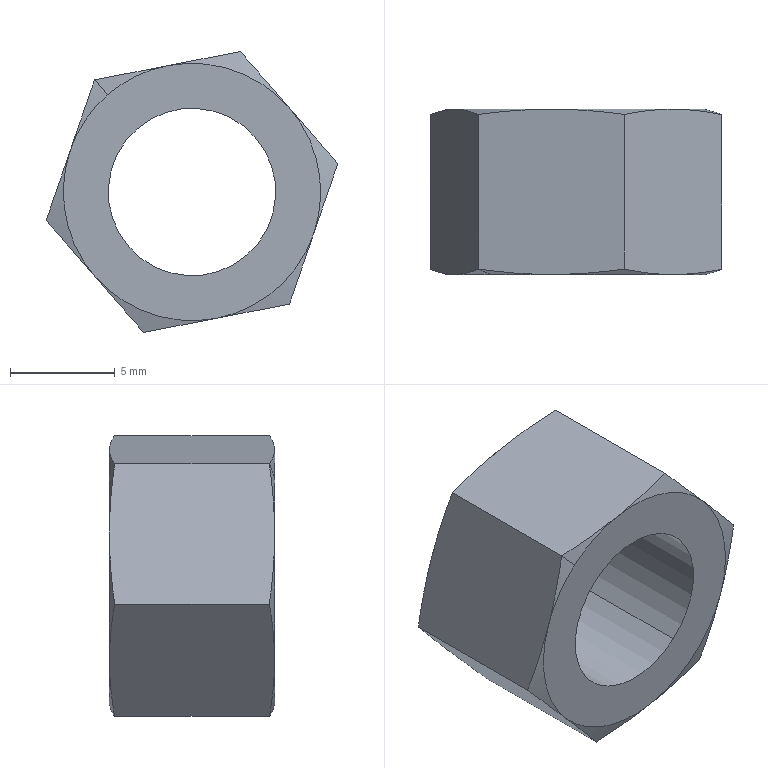Component | SolidWorks | GB_T41-2000Type1HexNutGradeCM8-1 | 1 solid | 24 faces | box 13.94 x 7.9 x 13.43 mm | volume 636 mm3 | cone 14 | plane 8 | cylinder 2 | commonest cylinder face diameters 8 x2
STEP:
#1=COLOUR_RGB('',0.7922,0.8196,0.9333);
#2=FILL_AREA_STYLE_COLOUR('',#1);
#3=FILL_AREA_STYLE('',(#2));
#4=SURFACE_STYLE_FILL_AREA(#3);
#5=SURFACE_SIDE_STYLE('',(#4));
#6=SURFACE_STYLE_USAGE(.BOTH.,#5);
#7=PRESENTATION_STYLE_ASSIGNMENT((#6));
#8=CARTESIAN_POINT('',(2.999,-2.205,10.51));
#9=VERTEX_POINT('',#8);
#10=CARTESIAN_POINT('',(3.112,-2.205,10.565));
#11=VERTEX_POINT('',#10);
#12=CARTESIAN_POINT('',(2.953,-2.205,10.748));
#13=DIRECTION('',(0.,-1.,-0.));
#14=DIRECTION('',(-0.656,-0.,0.7547));
#15=AXIS2_PLACEMENT_3D('',#12,#13,#14);
#16=CIRCLE('',#15,0.2421);
#17=EDGE_CURVE('',#9,#11,#16,.T.);
#18=ORIENTED_EDGE('',*,*,#17,.T.);
#19=CARTESIAN_POINT('',(3.136,-2.215,10.537));
#20=VERTEX_POINT('',#19);
#21=CARTESIAN_POINT('',(3.112,-2.205,10.565));
#22=DIRECTION('',(0.6337,-0.2588,-0.729));
#23=VECTOR('',#22,39.37);
#24=LINE('',#21,#23);
#25=EDGE_CURVE('',#11,#20,#24,.T.);
#26=ORIENTED_EDGE('',*,*,#25,.T.);
#27=CARTESIAN_POINT('',(3.136,-2.215,10.537));
#28=CARTESIAN_POINT('',(3.091,-2.209,10.528));
#29=CARTESIAN_POINT('',(3.045,-2.205,10.519));
#30=CARTESIAN_POINT('',(2.999,-2.205,10.51));
#31=B_SPLINE_CURVE_WITH_KNOTS('',3,(#27,#28,#29,#30),.UNSPECIFIED.,.F.,.F.,(4,4),(0.,0.003559),.UNSPECIFIED.);
#32=EDGE_CURVE('',#20,#9,#31,.T.);
#33=ORIENTED_EDGE('',*,*,#32,.T.);
#34=EDGE_LOOP('',(#18,#26,#33));
#35=FACE_OUTER_BOUND('',#34,.T.);
#36=CARTESIAN_POINT('',(2.953,-2.205,10.748));
#37=DIRECTION('',(0.,-1.,-0.));
#38=DIRECTION('',(0.656,0.,-0.7547));
#39=AXIS2_PLACEMENT_3D('',#36,#37,#38);
#40=CONICAL_SURFACE('',#39,0.2421,1.309);
#41=ADVANCED_FACE('',(#35),#40,.T.);
#42=CARTESIAN_POINT('',(2.794,-2.516,10.931));
#43=VERTEX_POINT('',#42);
#44=CARTESIAN_POINT('',(2.724,-2.516,10.827));
#45=VERTEX_POINT('',#44);
#46=CARTESIAN_POINT('',(2.953,-2.516,10.748));
#47=DIRECTION('',(0.,-1.,-0.));
#48=DIRECTION('',(-0.656,0.,0.7547));
#49=AXIS2_PLACEMENT_3D('',#46,#47,#48);
#50=CIRCLE('',#49,0.2421);
#51=EDGE_CURVE('',#43,#45,#50,.T.);
#52=ORIENTED_EDGE('',*,*,#51,.F.);
#53=CARTESIAN_POINT('',(2.769,-2.506,10.959));
#54=VERTEX_POINT('',#53);
#55=CARTESIAN_POINT('',(2.794,-2.516,10.931));
#56=DIRECTION('',(-0.6337,0.2588,0.729));
#57=VECTOR('',#56,39.37);
#58=LINE('',#55,#57);
#59=EDGE_CURVE('',#43,#54,#58,.T.);
#60=ORIENTED_EDGE('',*,*,#59,.T.);
#61=CARTESIAN_POINT('',(2.769,-2.506,10.959));
#62=CARTESIAN_POINT('',(2.754,-2.512,10.915));
#63=CARTESIAN_POINT('',(2.739,-2.516,10.871));
#64=CARTESIAN_POINT('',(2.724,-2.516,10.827));
#65=B_SPLINE_CURVE_WITH_KNOTS('',3,(#61,#62,#63,#64),.UNSPECIFIED.,.F.,.F.,(4,4),(0.,0.003559),.UNSPECIFIED.);
#66=EDGE_CURVE('',#54,#45,#65,.T.);
#67=ORIENTED_EDGE('',*,*,#66,.T.);
#68=EDGE_LOOP('',(#52,#60,#67));
#69=FACE_OUTER_BOUND('',#68,.T.);
#70=CARTESIAN_POINT('',(2.953,-2.516,10.748));
#71=DIRECTION('',(-0.,1.,0.));
#72=DIRECTION('',(-0.656,0.,0.7547));
#73=AXIS2_PLACEMENT_3D('',#70,#71,#72);
#74=CONICAL_SURFACE('',#73,0.2421,1.309);
#75=ADVANCED_FACE('',(#69),#74,.T.);
#76=CARTESIAN_POINT('',(2.849,-2.205,10.867));
#77=VERTEX_POINT('',#76);
#78=CARTESIAN_POINT('',(3.056,-2.205,10.629));
#79=VERTEX_POINT('',#78);
#80=CARTESIAN_POINT('',(2.953,-2.205,10.748));
#81=DIRECTION('',(-0.,1.,0.));
#82=DIRECTION('',(0.656,0.,-0.7547));
#83=AXIS2_PLACEMENT_3D('',#80,#81,#82);
#84=CIRCLE('',#83,0.1575);
#85=EDGE_CURVE('',#77,#79,#84,.T.);
#86=ORIENTED_EDGE('',*,*,#85,.T.);
#87=CARTESIAN_POINT('',(3.056,-2.516,10.629));
#88=VERTEX_POINT('',#87);
#89=CARTESIAN_POINT('',(3.056,-2.205,10.629));
#90=DIRECTION('',(0.,-1.,-0.));
#91=VECTOR('',#90,39.37);
#92=LINE('',#89,#91);
#93=EDGE_CURVE('',#79,#88,#92,.T.);
#94=ORIENTED_EDGE('',*,*,#93,.T.);
#95=CARTESIAN_POINT('',(2.849,-2.516,10.867));
#96=VERTEX_POINT('',#95);
#97=CARTESIAN_POINT('',(2.953,-2.516,10.748));
#98=DIRECTION('',(-0.,1.,0.));
#99=DIRECTION('',(0.656,0.,-0.7547));
#100=AXIS2_PLACEMENT_3D('',#97,#98,#99);
#101=CIRCLE('',#100,0.1575);
#102=EDGE_CURVE('',#96,#88,#101,.T.);
#103=ORIENTED_EDGE('',*,*,#102,.F.);
#104=CARTESIAN_POINT('',(2.849,-2.205,10.867));
#105=DIRECTION('',(0.,-1.,-0.));
#106=VECTOR('',#105,39.37);
#107=LINE('',#104,#106);
#108=EDGE_CURVE('',#77,#96,#107,.T.);
#109=ORIENTED_EDGE('',*,*,#108,.F.);
#110=EDGE_LOOP('',(#86,#94,#103,#109));
#111=FACE_OUTER_BOUND('',#110,.T.);
#112=CARTESIAN_POINT('',(2.953,-2.205,10.748));
#113=DIRECTION('',(0.,-1.,-0.));
#114=DIRECTION('',(-0.656,-0.,0.7547));
#115=AXIS2_PLACEMENT_3D('',#112,#113,#114);
#116=CYLINDRICAL_SURFACE('',#115,0.1575);
#117=ADVANCED_FACE('',(#111),#116,.F.);
#118=CARTESIAN_POINT('',(2.77,-2.205,10.589));
#119=VERTEX_POINT('',#118);
#120=CARTESIAN_POINT('',(2.678,-2.215,10.695));
#121=VERTEX_POINT('',#120);
#122=CARTESIAN_POINT('',(2.77,-2.205,10.589));
#123=CARTESIAN_POINT('',(2.739,-2.205,10.625));
#124=CARTESIAN_POINT('',(2.709,-2.209,10.66));
#125=CARTESIAN_POINT('',(2.678,-2.215,10.695));
#126=B_SPLINE_CURVE_WITH_KNOTS('',3,(#122,#123,#124,#125),.UNSPECIFIED.,.F.,.F.,(4,4),(0.,0.003559),.UNSPECIFIED.);
#127=EDGE_CURVE('',#119,#121,#126,.T.);
#128=ORIENTED_EDGE('',*,*,#127,.T.);
#129=CARTESIAN_POINT('',(2.724,-2.205,10.827));
#130=VERTEX_POINT('',#129);
#131=CARTESIAN_POINT('',(2.678,-2.215,10.695));
#132=CARTESIAN_POINT('',(2.693,-2.209,10.739));
#133=CARTESIAN_POINT('',(2.709,-2.205,10.783));
#134=CARTESIAN_POINT('',(2.724,-2.205,10.827));
#135=B_SPLINE_CURVE_WITH_KNOTS('',3,(#131,#132,#133,#134),.UNSPECIFIED.,.F.,.F.,(4,4),(0.,0.003559),.UNSPECIFIED.);
#136=EDGE_CURVE('',#121,#130,#135,.T.);
#137=ORIENTED_EDGE('',*,*,#136,.T.);
#138=CARTESIAN_POINT('',(2.953,-2.205,10.748));
#139=DIRECTION('',(0.,-1.,-0.));
#140=DIRECTION('',(-0.656,-0.,0.7547));
#141=AXIS2_PLACEMENT_3D('',#138,#139,#140);
#142=CIRCLE('',#141,0.2421);
#143=EDGE_CURVE('',#130,#119,#142,.T.);
#144=ORIENTED_EDGE('',*,*,#143,.T.);
#145=EDGE_LOOP('',(#128,#137,#144));
#146=FACE_OUTER_BOUND('',#145,.T.);
#147=CARTESIAN_POINT('',(2.953,-2.205,10.748));
#148=DIRECTION('',(0.,-1.,-0.));
#149=DIRECTION('',(0.656,0.,-0.7547));
#150=AXIS2_PLACEMENT_3D('',#147,#148,#149);
#151=CONICAL_SURFACE('',#150,0.2421,1.309);
#152=ADVANCED_FACE('',(#146),#151,.T.);
#153=CARTESIAN_POINT('',(2.862,-2.215,10.484));
#154=VERTEX_POINT('',#153);
#155=CARTESIAN_POINT('',(2.999,-2.205,10.51));
#156=CARTESIAN_POINT('',(2.953,-2.205,10.501));
#157=CARTESIAN_POINT('',(2.907,-2.209,10.493));
#158=CARTESIAN_POINT('',(2.862,-2.215,10.484));
#159=B_SPLINE_CURVE_WITH_KNOTS('',3,(#155,#156,#157,#158),.UNSPECIFIED.,.F.,.F.,(4,4),(0.,0.003559),.UNSPECIFIED.);
#160=EDGE_CURVE('',#9,#154,#159,.T.);
#161=ORIENTED_EDGE('',*,*,#160,.T.);
#162=CARTESIAN_POINT('',(2.862,-2.215,10.484));
#163=CARTESIAN_POINT('',(2.831,-2.209,10.519));
#164=CARTESIAN_POINT('',(2.801,-2.205,10.554));
#165=CARTESIAN_POINT('',(2.77,-2.205,10.589));
#166=B_SPLINE_CURVE_WITH_KNOTS('',3,(#162,#163,#164,#165),.UNSPECIFIED.,.F.,.F.,(4,4),(0.,0.003559),.UNSPECIFIED.);
#167=EDGE_CURVE('',#154,#119,#166,.T.);
#168=ORIENTED_EDGE('',*,*,#167,.T.);
#169=CARTESIAN_POINT('',(2.953,-2.205,10.748));
#170=DIRECTION('',(-0.,1.,0.));
#171=DIRECTION('',(0.656,0.,-0.7547));
#172=AXIS2_PLACEMENT_3D('',#169,#170,#171);
#173=CIRCLE('',#172,0.2421);
#174=EDGE_CURVE('',#9,#119,#173,.T.);
#175=ORIENTED_EDGE('',*,*,#174,.F.);
#176=EDGE_LOOP('',(#161,#168,#175));
#177=FACE_OUTER_BOUND('',#176,.T.);
#178=CARTESIAN_POINT('',(2.953,-2.205,10.748));
#179=DIRECTION('',(0.,-1.,-0.));
#180=DIRECTION('',(0.656,0.,-0.7547));
#181=AXIS2_PLACEMENT_3D('',#178,#179,#180);
#182=CONICAL_SURFACE('',#181,0.2421,1.309);
#183=ADVANCED_FACE('',(#177),#182,.T.);
#184=CARTESIAN_POINT('',(3.135,-2.205,10.907));
#185=VERTEX_POINT('',#184);
#186=CARTESIAN_POINT('',(3.227,-2.215,10.801));
#187=VERTEX_POINT('',#186);
#188=CARTESIAN_POINT('',(3.135,-2.205,10.907));
#189=CARTESIAN_POINT('',(3.166,-2.205,10.871));
#190=CARTESIAN_POINT('',(3.197,-2.209,10.836));
#191=CARTESIAN_POINT('',(3.227,-2.215,10.801));
#192=B_SPLINE_CURVE_WITH_KNOTS('',3,(#188,#189,#190,#191),.UNSPECIFIED.,.F.,.F.,(4,4),(0.,0.003559),.UNSPECIFIED.);
#193=EDGE_CURVE('',#185,#187,#192,.T.);
#194=ORIENTED_EDGE('',*,*,#193,.T.);
#195=CARTESIAN_POINT('',(3.182,-2.205,10.669));
#196=VERTEX_POINT('',#195);
#197=CARTESIAN_POINT('',(3.227,-2.215,10.801));
#198=CARTESIAN_POINT('',(3.212,-2.209,10.758));
#199=CARTESIAN_POINT('',(3.197,-2.205,10.713));
#200=CARTESIAN_POINT('',(3.182,-2.205,10.669));
#201=B_SPLINE_CURVE_WITH_KNOTS('',3,(#197,#198,#199,#200),.UNSPECIFIED.,.F.,.F.,(4,4),(0.,0.003559),.UNSPECIFIED.);
#202=EDGE_CURVE('',#187,#196,#201,.T.);
#203=ORIENTED_EDGE('',*,*,#202,.T.);
#204=CARTESIAN_POINT('',(2.953,-2.205,10.748));
#205=DIRECTION('',(0.,-1.,-0.));
#206=DIRECTION('',(-0.656,-0.,0.7547));
#207=AXIS2_PLACEMENT_3D('',#204,#205,#206);
#208=CIRCLE('',#207,0.2421);
#209=EDGE_CURVE('',#196,#185,#208,.T.);
#210=ORIENTED_EDGE('',*,*,#209,.T.);
#211=EDGE_LOOP('',(#194,#203,#210));
#212=FACE_OUTER_BOUND('',#211,.T.);
#213=CARTESIAN_POINT('',(2.953,-2.205,10.748));
#214=DIRECTION('',(0.,-1.,-0.));
#215=DIRECTION('',(0.656,0.,-0.7547));
#216=AXIS2_PLACEMENT_3D('',#213,#214,#215);
#217=CONICAL_SURFACE('',#216,0.2421,1.309);
#218=ADVANCED_FACE('',(#212),#217,.T.);
#219=CARTESIAN_POINT('',(2.907,-2.205,10.986));
#220=VERTEX_POINT('',#219);
#221=CARTESIAN_POINT('',(3.044,-2.215,11.012));
#222=VERTEX_POINT('',#221);
#223=CARTESIAN_POINT('',(2.907,-2.205,10.986));
#224=CARTESIAN_POINT('',(2.953,-2.205,10.995));
#225=CARTESIAN_POINT('',(2.998,-2.209,11.003));
#226=CARTESIAN_POINT('',(3.044,-2.215,11.012));
#227=B_SPLINE_CURVE_WITH_KNOTS('',3,(#223,#224,#225,#226),.UNSPECIFIED.,.F.,.F.,(4,4),(0.,0.003559),.UNSPECIFIED.);
#228=EDGE_CURVE('',#220,#222,#227,.T.);
#229=ORIENTED_EDGE('',*,*,#228,.T.);
#230=CARTESIAN_POINT('',(3.044,-2.215,11.012));
#231=CARTESIAN_POINT('',(3.074,-2.209,10.977));
#232=CARTESIAN_POINT('',(3.105,-2.205,10.942));
#233=CARTESIAN_POINT('',(3.135,-2.205,10.907));
#234=B_SPLINE_CURVE_WITH_KNOTS('',3,(#230,#231,#232,#233),.UNSPECIFIED.,.F.,.F.,(4,4),(0.,0.003559),.UNSPECIFIED.);
#235=EDGE_CURVE('',#222,#185,#234,.T.);
#236=ORIENTED_EDGE('',*,*,#235,.T.);
#237=CARTESIAN_POINT('',(2.953,-2.205,10.748));
#238=DIRECTION('',(0.,-1.,-0.));
#239=DIRECTION('',(-0.656,-0.,0.7547));
#240=AXIS2_PLACEMENT_3D('',#237,#238,#239);
#241=CIRCLE('',#240,0.2421);
#242=EDGE_CURVE('',#185,#220,#241,.T.);
#243=ORIENTED_EDGE('',*,*,#242,.T.);
#244=EDGE_LOOP('',(#229,#236,#243));
#245=FACE_OUTER_BOUND('',#244,.T.);
#246=CARTESIAN_POINT('',(2.953,-2.205,10.748));
#247=DIRECTION('',(0.,-1.,-0.));
#248=DIRECTION('',(0.656,0.,-0.7547));
#249=AXIS2_PLACEMENT_3D('',#246,#247,#248);
#250=CONICAL_SURFACE('',#249,0.2421,1.309);
#251=ADVANCED_FACE('',(#245),#250,.T.);
#252=CARTESIAN_POINT('',(2.769,-2.215,10.959));
#253=VERTEX_POINT('',#252);
#254=CARTESIAN_POINT('',(2.724,-2.205,10.827));
#255=CARTESIAN_POINT('',(2.739,-2.205,10.871));
#256=CARTESIAN_POINT('',(2.754,-2.209,10.915));
#257=CARTESIAN_POINT('',(2.769,-2.215,10.959));
#258=B_SPLINE_CURVE_WITH_KNOTS('',3,(#254,#255,#256,#257),.UNSPECIFIED.,.F.,.F.,(4,4),(0.,0.003559),.UNSPECIFIED.);
#259=EDGE_CURVE('',#130,#253,#258,.T.);
#260=ORIENTED_EDGE('',*,*,#259,.T.);
#261=CARTESIAN_POINT('',(2.769,-2.215,10.959));
#262=CARTESIAN_POINT('',(2.815,-2.209,10.968));
#263=CARTESIAN_POINT('',(2.861,-2.205,10.977));
#264=CARTESIAN_POINT('',(2.907,-2.205,10.986));
#265=B_SPLINE_CURVE_WITH_KNOTS('',3,(#261,#262,#263,#264),.UNSPECIFIED.,.F.,.F.,(4,4),(0.,0.003559),.UNSPECIFIED.);
#266=EDGE_CURVE('',#253,#220,#265,.T.);
#267=ORIENTED_EDGE('',*,*,#266,.T.);
#268=CARTESIAN_POINT('',(2.953,-2.205,10.748));
#269=DIRECTION('',(0.,-1.,-0.));
#270=DIRECTION('',(-0.656,-0.,0.7547));
#271=AXIS2_PLACEMENT_3D('',#268,#269,#270);
#272=CIRCLE('',#271,0.2421);
#273=EDGE_CURVE('',#220,#130,#272,.T.);
#274=ORIENTED_EDGE('',*,*,#273,.T.);
#275=EDGE_LOOP('',(#260,#267,#274));
#276=FACE_OUTER_BOUND('',#275,.T.);
#277=CARTESIAN_POINT('',(2.953,-2.205,10.748));
#278=DIRECTION('',(0.,-1.,-0.));
#279=DIRECTION('',(0.656,0.,-0.7547));
#280=AXIS2_PLACEMENT_3D('',#277,#278,#279);
#281=CONICAL_SURFACE('',#280,0.2421,1.309);
#282=ADVANCED_FACE('',(#276),#281,.T.);
#283=CARTESIAN_POINT('',(2.77,-2.516,10.589));
#284=VERTEX_POINT('',#283);
#285=CARTESIAN_POINT('',(2.862,-2.506,10.484));
#286=VERTEX_POINT('',#285);
#287=CARTESIAN_POINT('',(2.77,-2.516,10.589));
#288=CARTESIAN_POINT('',(2.801,-2.516,10.554));
#289=CARTESIAN_POINT('',(2.831,-2.512,10.519));
#290=CARTESIAN_POINT('',(2.862,-2.506,10.484));
#291=B_SPLINE_CURVE_WITH_KNOTS('',3,(#287,#288,#289,#290),.UNSPECIFIED.,.F.,.F.,(4,4),(0.,0.003559),.UNSPECIFIED.);
#292=EDGE_CURVE('',#284,#286,#291,.T.);
#293=ORIENTED_EDGE('',*,*,#292,.T.);
#294=CARTESIAN_POINT('',(2.999,-2.516,10.51));
#295=VERTEX_POINT('',#294);
#296=CARTESIAN_POINT('',(2.862,-2.506,10.484));
#297=CARTESIAN_POINT('',(2.907,-2.512,10.493));
#298=CARTESIAN_POINT('',(2.953,-2.516,10.501));
#299=CARTESIAN_POINT('',(2.999,-2.516,10.51));
#300=B_SPLINE_CURVE_WITH_KNOTS('',3,(#296,#297,#298,#299),.UNSPECIFIED.,.F.,.F.,(4,4),(0.,0.003559),.UNSPECIFIED.);
#301=EDGE_CURVE('',#286,#295,#300,.T.);
#302=ORIENTED_EDGE('',*,*,#301,.T.);
#303=CARTESIAN_POINT('',(2.953,-2.516,10.748));
#304=DIRECTION('',(0.,-1.,-0.));
#305=DIRECTION('',(-0.656,0.,0.7547));
#306=AXIS2_PLACEMENT_3D('',#303,#304,#305);
#307=CIRCLE('',#306,0.2421);
#308=EDGE_CURVE('',#284,#295,#307,.T.);
#309=ORIENTED_EDGE('',*,*,#308,.F.);
#310=EDGE_LOOP('',(#293,#302,#309));
#311=FACE_OUTER_BOUND('',#310,.T.);
#312=CARTESIAN_POINT('',(2.953,-2.516,10.748));
#313=DIRECTION('',(-0.,1.,0.));
#314=DIRECTION('',(-0.656,0.,0.7547));
#315=AXIS2_PLACEMENT_3D('',#312,#313,#314);
#316=CONICAL_SURFACE('',#315,0.2421,1.309);
#317=ADVANCED_FACE('',(#311),#316,.T.);
#318=CARTESIAN_POINT('',(2.678,-2.506,10.695));
#319=VERTEX_POINT('',#318);
#320=CARTESIAN_POINT('',(2.724,-2.516,10.827));
#321=CARTESIAN_POINT('',(2.709,-2.516,10.783));
#322=CARTESIAN_POINT('',(2.693,-2.512,10.739));
#323=CARTESIAN_POINT('',(2.678,-2.506,10.695));
#324=B_SPLINE_CURVE_WITH_KNOTS('',3,(#320,#321,#322,#323),.UNSPECIFIED.,.F.,.F.,(4,4),(0.,0.003559),.UNSPECIFIED.);
#325=EDGE_CURVE('',#45,#319,#324,.T.);
#326=ORIENTED_EDGE('',*,*,#325,.T.);
#327=CARTESIAN_POINT('',(2.678,-2.506,10.695));
#328=CARTESIAN_POINT('',(2.709,-2.512,10.66));
#329=CARTESIAN_POINT('',(2.739,-2.516,10.625));
#330=CARTESIAN_POINT('',(2.77,-2.516,10.589));
#331=B_SPLINE_CURVE_WITH_KNOTS('',3,(#327,#328,#329,#330),.UNSPECIFIED.,.F.,.F.,(4,4),(0.,0.003559),.UNSPECIFIED.);
#332=EDGE_CURVE('',#319,#284,#331,.T.);
#333=ORIENTED_EDGE('',*,*,#332,.T.);
#334=CARTESIAN_POINT('',(2.953,-2.516,10.748));
#335=DIRECTION('',(0.,-1.,-0.));
#336=DIRECTION('',(-0.656,0.,0.7547));
#337=AXIS2_PLACEMENT_3D('',#334,#335,#336);
#338=CIRCLE('',#337,0.2421);
#339=EDGE_CURVE('',#45,#284,#338,.T.);
#340=ORIENTED_EDGE('',*,*,#339,.F.);
#341=EDGE_LOOP('',(#326,#333,#340));
#342=FACE_OUTER_BOUND('',#341,.T.);
#343=CARTESIAN_POINT('',(2.953,-2.516,10.748));
#344=DIRECTION('',(-0.,1.,0.));
#345=DIRECTION('',(-0.656,0.,0.7547));
#346=AXIS2_PLACEMENT_3D('',#343,#344,#345);
#347=CONICAL_SURFACE('',#346,0.2421,1.309);
#348=ADVANCED_FACE('',(#342),#347,.T.);
#349=CARTESIAN_POINT('',(3.044,-2.506,11.012));
#350=VERTEX_POINT('',#349);
#351=CARTESIAN_POINT('',(2.907,-2.516,10.986));
#352=VERTEX_POINT('',#351);
#353=CARTESIAN_POINT('',(3.044,-2.506,11.012));
#354=CARTESIAN_POINT('',(2.998,-2.512,11.003));
#355=CARTESIAN_POINT('',(2.953,-2.516,10.995));
#356=CARTESIAN_POINT('',(2.907,-2.516,10.986));
#357=B_SPLINE_CURVE_WITH_KNOTS('',3,(#353,#354,#355,#356),.UNSPECIFIED.,.F.,.F.,(4,4),(0.,0.003559),.UNSPECIFIED.);
#358=EDGE_CURVE('',#350,#352,#357,.T.);
#359=ORIENTED_EDGE('',*,*,#358,.T.);
#360=CARTESIAN_POINT('',(3.135,-2.516,10.907));
#361=VERTEX_POINT('',#360);
#362=CARTESIAN_POINT('',(2.953,-2.516,10.748));
#363=DIRECTION('',(0.,-1.,-0.));
#364=DIRECTION('',(-0.656,0.,0.7547));
#365=AXIS2_PLACEMENT_3D('',#362,#363,#364);
#366=CIRCLE('',#365,0.2421);
#367=EDGE_CURVE('',#361,#352,#366,.T.);
#368=ORIENTED_EDGE('',*,*,#367,.F.);
#369=CARTESIAN_POINT('',(3.135,-2.516,10.907));
#370=CARTESIAN_POINT('',(3.105,-2.516,10.942));
#371=CARTESIAN_POINT('',(3.074,-2.512,10.977));
#372=CARTESIAN_POINT('',(3.044,-2.506,11.012));
#373=B_SPLINE_CURVE_WITH_KNOTS('',3,(#369,#370,#371,#372),.UNSPECIFIED.,.F.,.F.,(4,4),(0.,0.003559),.UNSPECIFIED.);
#374=EDGE_CURVE('',#361,#350,#373,.T.);
#375=ORIENTED_EDGE('',*,*,#374,.T.);
#376=EDGE_LOOP('',(#359,#368,#375));
#377=FACE_OUTER_BOUND('',#376,.T.);
#378=CARTESIAN_POINT('',(2.953,-2.516,10.748));
#379=DIRECTION('',(-0.,1.,0.));
#380=DIRECTION('',(-0.656,0.,0.7547));
#381=AXIS2_PLACEMENT_3D('',#378,#379,#380);
#382=CONICAL_SURFACE('',#381,0.2421,1.309);
#383=ADVANCED_FACE('',(#377),#382,.T.);
#384=CARTESIAN_POINT('',(3.136,-2.506,10.537));
#385=VERTEX_POINT('',#384);
#386=CARTESIAN_POINT('',(2.999,-2.516,10.51));
#387=CARTESIAN_POINT('',(3.045,-2.516,10.519));
#388=CARTESIAN_POINT('',(3.091,-2.512,10.528));
#389=CARTESIAN_POINT('',(3.136,-2.506,10.537));
#390=B_SPLINE_CURVE_WITH_KNOTS('',3,(#386,#387,#388,#389),.UNSPECIFIED.,.F.,.F.,(4,4),(0.,0.003559),.UNSPECIFIED.);
#391=EDGE_CURVE('',#295,#385,#390,.T.);
#392=ORIENTED_EDGE('',*,*,#391,.T.);
#393=CARTESIAN_POINT('',(3.182,-2.516,10.669));
#394=VERTEX_POINT('',#393);
#395=CARTESIAN_POINT('',(3.136,-2.506,10.537));
#396=CARTESIAN_POINT('',(3.151,-2.512,10.581));
#397=CARTESIAN_POINT('',(3.166,-2.516,10.625));
#398=CARTESIAN_POINT('',(3.182,-2.516,10.669));
#399=B_SPLINE_CURVE_WITH_KNOTS('',3,(#395,#396,#397,#398),.UNSPECIFIED.,.F.,.F.,(4,4),(0.,0.003559),.UNSPECIFIED.);
#400=EDGE_CURVE('',#385,#394,#399,.T.);
#401=ORIENTED_EDGE('',*,*,#400,.T.);
#402=CARTESIAN_POINT('',(2.953,-2.516,10.748));
#403=DIRECTION('',(0.,-1.,-0.));
#404=DIRECTION('',(-0.656,0.,0.7547));
#405=AXIS2_PLACEMENT_3D('',#402,#403,#404);
#406=CIRCLE('',#405,0.2421);
#407=EDGE_CURVE('',#295,#394,#406,.T.);
#408=ORIENTED_EDGE('',*,*,#407,.F.);
#409=EDGE_LOOP('',(#392,#401,#408));
#410=FACE_OUTER_BOUND('',#409,.T.);
#411=CARTESIAN_POINT('',(2.953,-2.516,10.748));
#412=DIRECTION('',(-0.,1.,0.));
#413=DIRECTION('',(-0.656,0.,0.7547));
#414=AXIS2_PLACEMENT_3D('',#411,#412,#413);
#415=CONICAL_SURFACE('',#414,0.2421,1.309);
#416=ADVANCED_FACE('',(#410),#415,.T.);
#417=CARTESIAN_POINT('',(3.227,-2.506,10.801));
#418=VERTEX_POINT('',#417);
#419=CARTESIAN_POINT('',(3.227,-2.506,10.801));
#420=CARTESIAN_POINT('',(3.197,-2.512,10.836));
#421=CARTESIAN_POINT('',(3.166,-2.516,10.871));
#422=CARTESIAN_POINT('',(3.135,-2.516,10.907));
#423=B_SPLINE_CURVE_WITH_KNOTS('',3,(#419,#420,#421,#422),.UNSPECIFIED.,.F.,.F.,(4,4),(0.,0.003559),.UNSPECIFIED.);
#424=EDGE_CURVE('',#418,#361,#423,.T.);
#425=ORIENTED_EDGE('',*,*,#424,.T.);
#426=CARTESIAN_POINT('',(2.953,-2.516,10.748));
#427=DIRECTION('',(0.,-1.,-0.));
#428=DIRECTION('',(-0.656,0.,0.7547));
#429=AXIS2_PLACEMENT_3D('',#426,#427,#428);
#430=CIRCLE('',#429,0.2421);
#431=EDGE_CURVE('',#394,#361,#430,.T.);
#432=ORIENTED_EDGE('',*,*,#431,.F.);
#433=CARTESIAN_POINT('',(3.182,-2.516,10.669));
#434=CARTESIAN_POINT('',(3.197,-2.516,10.713));
#435=CARTESIAN_POINT('',(3.212,-2.512,10.758));
#436=CARTESIAN_POINT('',(3.227,-2.506,10.801));
#437=B_SPLINE_CURVE_WITH_KNOTS('',3,(#433,#434,#435,#436),.UNSPECIFIED.,.F.,.F.,(4,4),(0.,0.003559),.UNSPECIFIED.);
#438=EDGE_CURVE('',#394,#418,#437,.T.);
#439=ORIENTED_EDGE('',*,*,#438,.T.);
#440=EDGE_LOOP('',(#425,#432,#439));
#441=FACE_OUTER_BOUND('',#440,.T.);
#442=CARTESIAN_POINT('',(2.953,-2.516,10.748));
#443=DIRECTION('',(-0.,1.,0.));
#444=DIRECTION('',(-0.656,0.,0.7547));
#445=AXIS2_PLACEMENT_3D('',#442,#443,#444);
#446=CONICAL_SURFACE('',#445,0.2421,1.309);
#447=ADVANCED_FACE('',(#441),#446,.T.);
#448=ORIENTED_EDGE('',*,*,#102,.T.);
#449=CARTESIAN_POINT('',(2.953,-2.516,10.748));
#450=DIRECTION('',(-0.,1.,0.));
#451=DIRECTION('',(0.656,0.,-0.7547));
#452=AXIS2_PLACEMENT_3D('',#449,#450,#451);
#453=CIRCLE('',#452,0.1575);
#454=EDGE_CURVE('',#88,#96,#453,.T.);
#455=ORIENTED_EDGE('',*,*,#454,.T.);
#456=EDGE_LOOP('',(#448,#455));
#457=FACE_BOUND('',#456,.T.);
#458=ORIENTED_EDGE('',*,*,#367,.T.);
#459=CARTESIAN_POINT('',(2.953,-2.516,10.748));
#460=DIRECTION('',(0.,-1.,-0.));
#461=DIRECTION('',(-0.656,0.,0.7547));
#462=AXIS2_PLACEMENT_3D('',#459,#460,#461);
#463=CIRCLE('',#462,0.2421);
#464=EDGE_CURVE('',#352,#43,#463,.T.);
#465=ORIENTED_EDGE('',*,*,#464,.T.);
#466=ORIENTED_EDGE('',*,*,#51,.T.);
#467=ORIENTED_EDGE('',*,*,#339,.T.);
#468=ORIENTED_EDGE('',*,*,#308,.T.);
#469=ORIENTED_EDGE('',*,*,#407,.T.);
#470=ORIENTED_EDGE('',*,*,#431,.T.);
#471=EDGE_LOOP('',(#458,#465,#466,#467,#468,#469,#470));
#472=FACE_OUTER_BOUND('',#471,.T.);
#473=CARTESIAN_POINT('',(3.411,-2.516,10.59));
#474=DIRECTION('',(0.,-1.,-0.));
#475=DIRECTION('',(0.7547,0.,0.656));
#476=AXIS2_PLACEMENT_3D('',#473,#474,#475);
#477=PLANE('',#476);
#478=ADVANCED_FACE('',(#457,#472),#477,.T.);
#479=ORIENTED_EDGE('',*,*,#85,.F.);
#480=CARTESIAN_POINT('',(2.953,-2.205,10.748));
#481=DIRECTION('',(-0.,1.,0.));
#482=DIRECTION('',(0.656,0.,-0.7547));
#483=AXIS2_PLACEMENT_3D('',#480,#481,#482);
#484=CIRCLE('',#483,0.1575);
#485=EDGE_CURVE('',#79,#77,#484,.T.);
#486=ORIENTED_EDGE('',*,*,#485,.F.);
#487=EDGE_LOOP('',(#479,#486));
#488=FACE_BOUND('',#487,.T.);
#489=ORIENTED_EDGE('',*,*,#143,.F.);
#490=ORIENTED_EDGE('',*,*,#273,.F.);
#491=ORIENTED_EDGE('',*,*,#242,.F.);
#492=ORIENTED_EDGE('',*,*,#209,.F.);
#493=CARTESIAN_POINT('',(2.953,-2.205,10.748));
#494=DIRECTION('',(0.,-1.,-0.));
#495=DIRECTION('',(-0.656,-0.,0.7547));
#496=AXIS2_PLACEMENT_3D('',#493,#494,#495);
#497=CIRCLE('',#496,0.2421);
#498=EDGE_CURVE('',#11,#196,#497,.T.);
#499=ORIENTED_EDGE('',*,*,#498,.F.);
#500=ORIENTED_EDGE('',*,*,#17,.F.);
#501=ORIENTED_EDGE('',*,*,#174,.T.);
#502=EDGE_LOOP('',(#489,#490,#491,#492,#499,#500,#501));
#503=FACE_OUTER_BOUND('',#502,.T.);
#504=CARTESIAN_POINT('',(3.411,-2.205,10.59));
#505=DIRECTION('',(0.,-1.,-0.));
#506=DIRECTION('',(0.7547,0.,0.656));
#507=AXIS2_PLACEMENT_3D('',#504,#505,#506);
#508=PLANE('',#507);
#509=ADVANCED_FACE('',(#488,#503),#508,.F.);
#510=ORIENTED_EDGE('',*,*,#202,.F.);
#511=CARTESIAN_POINT('',(3.227,-2.205,10.801));
#512=DIRECTION('',(0.,-1.,-0.));
#513=VECTOR('',#512,39.37);
#514=LINE('',#511,#513);
#515=EDGE_CURVE('',#187,#418,#514,.T.);
#516=ORIENTED_EDGE('',*,*,#515,.T.);
#517=ORIENTED_EDGE('',*,*,#438,.F.);
#518=ORIENTED_EDGE('',*,*,#400,.F.);
#519=CARTESIAN_POINT('',(3.136,-2.205,10.537));
#520=DIRECTION('',(0.,-1.,-0.));
#521=VECTOR('',#520,39.37);
#522=LINE('',#519,#521);
#523=EDGE_CURVE('',#20,#385,#522,.T.);
#524=ORIENTED_EDGE('',*,*,#523,.F.);
#525=CARTESIAN_POINT('',(3.182,-2.205,10.669));
#526=CARTESIAN_POINT('',(3.166,-2.205,10.625));
#527=CARTESIAN_POINT('',(3.151,-2.209,10.581));
#528=CARTESIAN_POINT('',(3.136,-2.215,10.537));
#529=B_SPLINE_CURVE_WITH_KNOTS('',3,(#525,#526,#527,#528),.UNSPECIFIED.,.F.,.F.,(4,4),(0.,0.003559),.UNSPECIFIED.);
#530=EDGE_CURVE('',#196,#20,#529,.T.);
#531=ORIENTED_EDGE('',*,*,#530,.F.);
#532=EDGE_LOOP('',(#510,#516,#517,#518,#524,#531));
#533=FACE_OUTER_BOUND('',#532,.T.);
#534=CARTESIAN_POINT('',(3.227,-2.205,10.801));
#535=DIRECTION('',(-0.9455,-0.,0.3256));
#536=DIRECTION('',(-0.,1.,0.));
#537=AXIS2_PLACEMENT_3D('',#534,#535,#536);
#538=PLANE('',#537);
#539=ADVANCED_FACE('',(#533),#538,.F.);
#540=ORIENTED_EDGE('',*,*,#235,.F.);
#541=CARTESIAN_POINT('',(3.044,-2.205,11.012));
#542=DIRECTION('',(0.,-1.,-0.));
#543=VECTOR('',#542,39.37);
#544=LINE('',#541,#543);
#545=EDGE_CURVE('',#222,#350,#544,.T.);
#546=ORIENTED_EDGE('',*,*,#545,.T.);
#547=ORIENTED_EDGE('',*,*,#374,.F.);
#548=ORIENTED_EDGE('',*,*,#424,.F.);
#549=ORIENTED_EDGE('',*,*,#515,.F.);
#550=ORIENTED_EDGE('',*,*,#193,.F.);
#551=EDGE_LOOP('',(#540,#546,#547,#548,#549,#550));
#552=FACE_OUTER_BOUND('',#551,.T.);
#553=CARTESIAN_POINT('',(3.044,-2.205,11.012));
#554=DIRECTION('',(-0.7547,0.,-0.656));
#555=DIRECTION('',(0.656,0.,-0.7547));
#556=AXIS2_PLACEMENT_3D('',#553,#554,#555);
#557=PLANE('',#556);
#558=ADVANCED_FACE('',(#552),#557,.F.);
#559=ORIENTED_EDGE('',*,*,#266,.F.);
#560=CARTESIAN_POINT('',(2.769,-2.205,10.959));
#561=DIRECTION('',(0.,-1.,-0.));
#562=VECTOR('',#561,39.37);
#563=LINE('',#560,#562);
#564=EDGE_CURVE('',#253,#54,#563,.T.);
#565=ORIENTED_EDGE('',*,*,#564,.T.);
#566=CARTESIAN_POINT('',(2.907,-2.516,10.986));
#567=CARTESIAN_POINT('',(2.861,-2.516,10.977));
#568=CARTESIAN_POINT('',(2.815,-2.512,10.968));
#569=CARTESIAN_POINT('',(2.769,-2.506,10.959));
#570=B_SPLINE_CURVE_WITH_KNOTS('',3,(#566,#567,#568,#569),.UNSPECIFIED.,.F.,.F.,(4,4),(0.,0.003559),.UNSPECIFIED.);
#571=EDGE_CURVE('',#352,#54,#570,.T.);
#572=ORIENTED_EDGE('',*,*,#571,.F.);
#573=ORIENTED_EDGE('',*,*,#358,.F.);
#574=ORIENTED_EDGE('',*,*,#545,.F.);
#575=ORIENTED_EDGE('',*,*,#228,.F.);
#576=EDGE_LOOP('',(#559,#565,#572,#573,#574,#575));
#577=FACE_OUTER_BOUND('',#576,.T.);
#578=CARTESIAN_POINT('',(2.769,-2.205,10.959));
#579=DIRECTION('',(0.1908,0.,-0.9816));
#580=DIRECTION('',(0.,-1.,-0.));
#581=AXIS2_PLACEMENT_3D('',#578,#579,#580);
#582=PLANE('',#581);
#583=ADVANCED_FACE('',(#577),#582,.F.);
#584=ORIENTED_EDGE('',*,*,#136,.F.);
#585=CARTESIAN_POINT('',(2.678,-2.205,10.695));
#586=DIRECTION('',(0.,-1.,-0.));
#587=VECTOR('',#586,39.37);
#588=LINE('',#585,#587);
#589=EDGE_CURVE('',#121,#319,#588,.T.);
#590=ORIENTED_EDGE('',*,*,#589,.T.);
#591=ORIENTED_EDGE('',*,*,#325,.F.);
#592=ORIENTED_EDGE('',*,*,#66,.F.);
#593=ORIENTED_EDGE('',*,*,#564,.F.);
#594=ORIENTED_EDGE('',*,*,#259,.F.);
#595=EDGE_LOOP('',(#584,#590,#591,#592,#593,#594));
#596=FACE_OUTER_BOUND('',#595,.T.);
#597=CARTESIAN_POINT('',(2.678,-2.205,10.695));
#598=DIRECTION('',(0.9455,0.,-0.3256));
#599=DIRECTION('',(0.,-1.,-0.));
#600=AXIS2_PLACEMENT_3D('',#597,#598,#599);
#601=PLANE('',#600);
#602=ADVANCED_FACE('',(#596),#601,.F.);
#603=ORIENTED_EDGE('',*,*,#167,.F.);
#604=CARTESIAN_POINT('',(2.862,-2.205,10.484));
#605=DIRECTION('',(0.,-1.,-0.));
#606=VECTOR('',#605,39.37);
#607=LINE('',#604,#606);
#608=EDGE_CURVE('',#154,#286,#607,.T.);
#609=ORIENTED_EDGE('',*,*,#608,.T.);
#610=ORIENTED_EDGE('',*,*,#292,.F.);
#611=ORIENTED_EDGE('',*,*,#332,.F.);
#612=ORIENTED_EDGE('',*,*,#589,.F.);
#613=ORIENTED_EDGE('',*,*,#127,.F.);
#614=EDGE_LOOP('',(#603,#609,#610,#611,#612,#613));
#615=FACE_OUTER_BOUND('',#614,.T.);
#616=CARTESIAN_POINT('',(2.862,-2.205,10.484));
#617=DIRECTION('',(0.7547,0.,0.656));
#618=DIRECTION('',(0.,-1.,-0.));
#619=AXIS2_PLACEMENT_3D('',#616,#617,#618);
#620=PLANE('',#619);
#621=ADVANCED_FACE('',(#615),#620,.F.);
#622=ORIENTED_EDGE('',*,*,#32,.F.);
#623=ORIENTED_EDGE('',*,*,#523,.T.);
#624=ORIENTED_EDGE('',*,*,#391,.F.);
#625=ORIENTED_EDGE('',*,*,#301,.F.);
#626=ORIENTED_EDGE('',*,*,#608,.F.);
#627=ORIENTED_EDGE('',*,*,#160,.F.);
#628=EDGE_LOOP('',(#622,#623,#624,#625,#626,#627));
#629=FACE_OUTER_BOUND('',#628,.T.);
#630=CARTESIAN_POINT('',(3.136,-2.205,10.537));
#631=DIRECTION('',(-0.1908,-0.,0.9816));
#632=DIRECTION('',(-0.9816,-0.,-0.1908));
#633=AXIS2_PLACEMENT_3D('',#630,#631,#632);
#634=PLANE('',#633);
#635=ADVANCED_FACE('',(#629),#634,.F.);
#636=ORIENTED_EDGE('',*,*,#93,.F.);
#637=ORIENTED_EDGE('',*,*,#485,.T.);
#638=ORIENTED_EDGE('',*,*,#108,.T.);
#639=ORIENTED_EDGE('',*,*,#454,.F.);
#640=EDGE_LOOP('',(#636,#637,#638,#639));
#641=FACE_OUTER_BOUND('',#640,.T.);
#642=CARTESIAN_POINT('',(2.953,-2.205,10.748));
#643=DIRECTION('',(0.,-1.,-0.));
#644=DIRECTION('',(-0.656,-0.,0.7547));
#645=AXIS2_PLACEMENT_3D('',#642,#643,#644);
#646=CYLINDRICAL_SURFACE('',#645,0.1575);
#647=ADVANCED_FACE('',(#641),#646,.F.);
#648=ORIENTED_EDGE('',*,*,#59,.F.);
#649=ORIENTED_EDGE('',*,*,#464,.F.);
#650=ORIENTED_EDGE('',*,*,#571,.T.);
#651=EDGE_LOOP('',(#648,#649,#650));
#652=FACE_OUTER_BOUND('',#651,.T.);
#653=CARTESIAN_POINT('',(2.953,-2.516,10.748));
#654=DIRECTION('',(-0.,1.,0.));
#655=DIRECTION('',(-0.656,0.,0.7547));
#656=AXIS2_PLACEMENT_3D('',#653,#654,#655);
#657=CONICAL_SURFACE('',#656,0.2421,1.309);
#658=ADVANCED_FACE('',(#652),#657,.T.);
#659=ORIENTED_EDGE('',*,*,#25,.F.);
#660=ORIENTED_EDGE('',*,*,#498,.T.);
#661=ORIENTED_EDGE('',*,*,#530,.T.);
#662=EDGE_LOOP('',(#659,#660,#661));
#663=FACE_OUTER_BOUND('',#662,.T.);
#664=CARTESIAN_POINT('',(2.953,-2.205,10.748));
#665=DIRECTION('',(0.,-1.,-0.));
#666=DIRECTION('',(0.656,0.,-0.7547));
#667=AXIS2_PLACEMENT_3D('',#664,#665,#666);
#668=CONICAL_SURFACE('',#667,0.2421,1.309);
#669=ADVANCED_FACE('',(#663),#668,.T.);
#670=CLOSED_SHELL('',(#41,#75,#117,#152,#183,#218,#251,#282,#317,#348,#383,#416,#447,#478,#509,#539,#558,#583,#602,#621,#635,#647,#658,#669));
#671=MANIFOLD_SOLID_BREP('',#670);
#672=STYLED_ITEM('',(#7),#671);
#673=PRESENTATION_LAYER_ASSIGNMENT('','',(#672));
#674=(LENGTH_UNIT()NAMED_UNIT(*)SI_UNIT($,.METRE.));
#675=LENGTH_MEASURE_WITH_UNIT(LENGTH_MEASURE(0.0254),#674);
#676=DIMENSIONAL_EXPONENTS(1.,0.,0.,0.,0.,0.,0.);
#677=(CONVERSION_BASED_UNIT('',#675)LENGTH_UNIT()NAMED_UNIT(#676));
#678=UNCERTAINTY_MEASURE_WITH_UNIT(LENGTH_MEASURE(0.00001),#677,'','');
#679=(NAMED_UNIT(*)PLANE_ANGLE_UNIT()SI_UNIT($,.RADIAN.));
#680=(NAMED_UNIT(*)SI_UNIT($,.STERADIAN.)SOLID_ANGLE_UNIT());
#681=(GEOMETRIC_REPRESENTATION_CONTEXT(3)GLOBAL_UNCERTAINTY_ASSIGNED_CONTEXT((#678))GLOBAL_UNIT_ASSIGNED_CONTEXT((#677,#679,#680))REPRESENTATION_CONTEXT('',''));
#682=MECHANICAL_DESIGN_GEOMETRIC_PRESENTATION_REPRESENTATION('',(#672),#681);
#683=CARTESIAN_POINT('',(0.,0.,0.));
#684=DIRECTION('',(0.,0.,1.));
#685=DIRECTION('',(1.,0.,0.));
#686=AXIS2_PLACEMENT_3D('',#683,#684,#685);
#687=(LENGTH_UNIT()NAMED_UNIT(*)SI_UNIT($,.METRE.));
#688=LENGTH_MEASURE_WITH_UNIT(LENGTH_MEASURE(0.0254),#687);
#689=DIMENSIONAL_EXPONENTS(1.,0.,0.,0.,0.,0.,0.);
#690=(CONVERSION_BASED_UNIT('',#688)LENGTH_UNIT()NAMED_UNIT(#689));
#691=UNCERTAINTY_MEASURE_WITH_UNIT(LENGTH_MEASURE(0.00001),#690,'','');
#692=(NAMED_UNIT(*)PLANE_ANGLE_UNIT()SI_UNIT($,.RADIAN.));
#693=(NAMED_UNIT(*)SI_UNIT($,.STERADIAN.)SOLID_ANGLE_UNIT());
#694=(GEOMETRIC_REPRESENTATION_CONTEXT(3)GLOBAL_UNCERTAINTY_ASSIGNED_CONTEXT((#691))GLOBAL_UNIT_ASSIGNED_CONTEXT((#690,#692,#693))REPRESENTATION_CONTEXT('',''));
#695=ADVANCED_BREP_SHAPE_REPRESENTATION('',(#671,#686),#694);